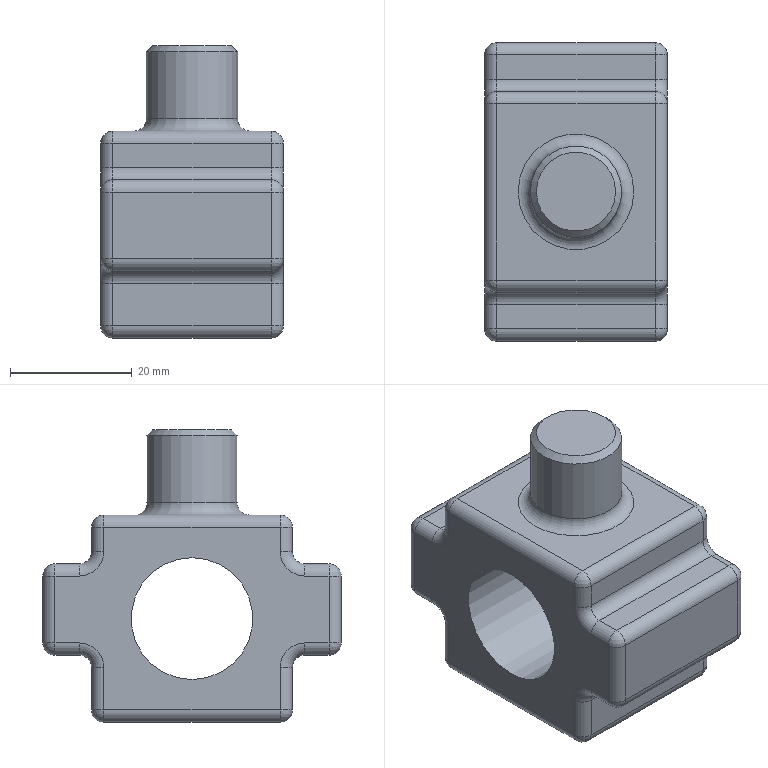Component | NX | NUT_2 | 1 solid | 79 faces | volume 33564 mm3 | cylinder 38 | sphere 16 | plane 15 | torus 9 | cone 1 | commonest cylinder face diameters 4 x36 15 x1 20 x1